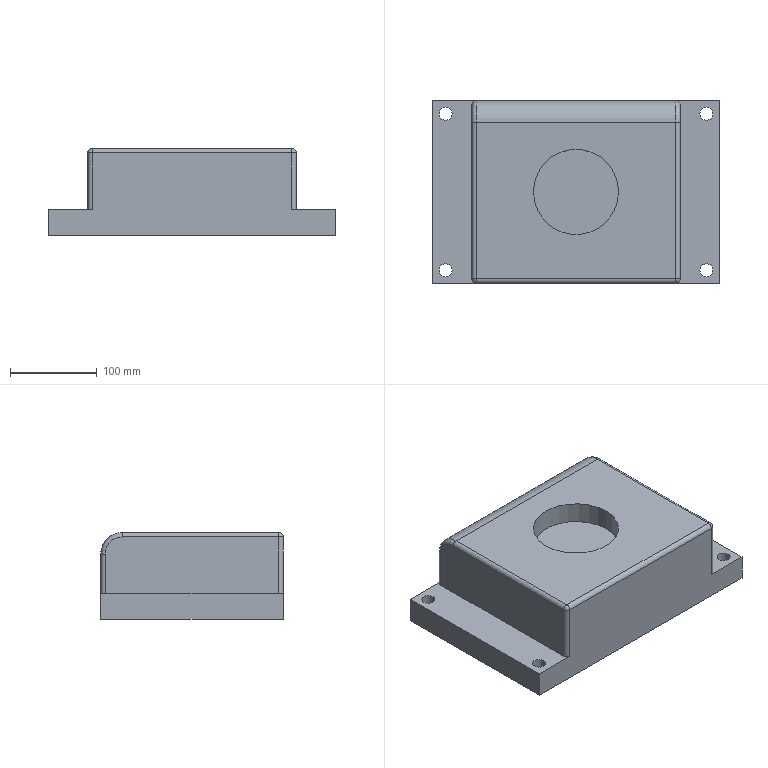Component | NX | M1002_AGO13_P09_A00757058_P03 | 1 solid | 28 faces | volume 5360163 mm3 | cylinder 13 | plane 11 | torus 2 | sphere 2 | commonest cylinder face diameters 10 x7 15 x4 98 x1 50 x1